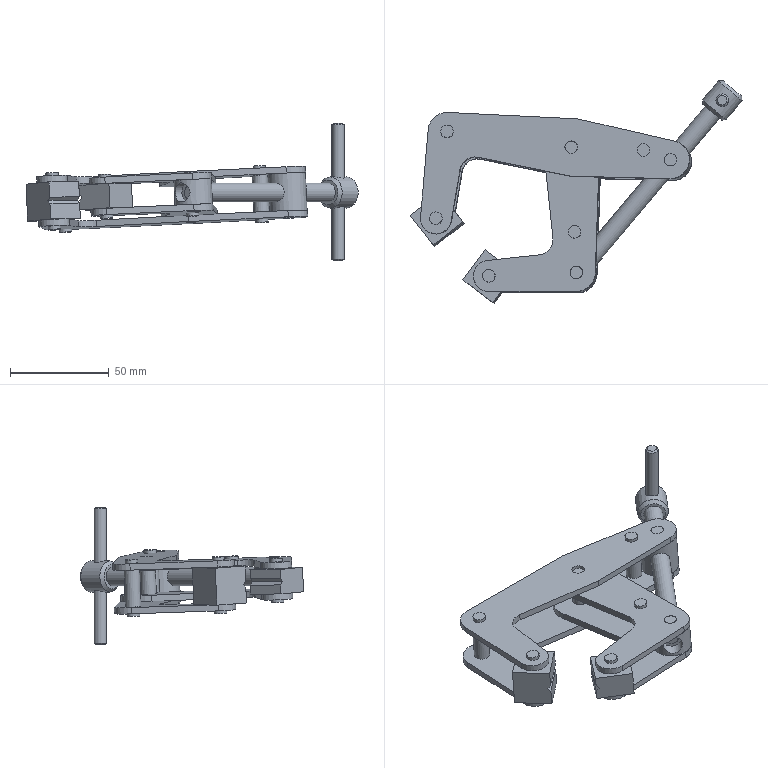Assembly | NX | mm | 16 component files | 16 solids | 158 faces | box 168.42 x 113.11 x 69.85 mm | volume 74950 mm3 | plane 86 | cylinder 68 | cone 4 | commonest cylinder face diameters 6.35 x36 15.748 x9 7.874 x8 19.304 x6 9.525 x2 28.448 x2 7.925 x2 19.05 x2
Bill of materials:
unnamed part 1 | 3 |  | Stepped cylindrical pin: one larger-diameter central body with a smaller coaxial journal at each end.
unnamed part 2 | 1 |  | Roughly cube-shaped rectangular block with a round through hole across one axis and a V-shaped groove running across one side face.
unnamed part 3 | 1 |  | Rectangular block with a round through hole and a single V-shaped notch along one edge face. It looks similar to the other grooved block but with different proportions or groove position.
unnamed part 4 | 2 |  | Flat plate shaped like a dog-leg or L in plan, with rounded ends and five round through holes spread along its arms.
unnamed part 5 | 1 |  | Plain slender solid cylindrical pin or rod with small chamfers at both ends.
unnamed part 6 | 1 |  | Short cylindrical body with one flat cut along its side, a cross hole through it at right angles to the axis, and small coaxial bosses at both ends.
unnamed part 7 | 2 |  | Flat L-shaped plate with rounded ends and corners and four round through holes.
unnamed part 8 | 3 |  | Stepped cylindrical pin with a larger central body and smaller coaxial journals at both ends. It is very similar to the other stepped pin.
unnamed part 9 | 1 |  | Long cylindrical shaft with a larger cylindrical head at one end that has a cross hole through it. The other end steps down to a smaller-diameter tip.
unnamed part 10 | 1 |  | Short cylindrical body with a plain round cross hole through it at right angles to the axis and small coaxial cylindrical bosses at both ends.
Mates:
1. concentric | Riostra_A 2 edge | Riostra_B 2 edge
2. concentric | Pasador_A 3 edge | Riostra_A 2 edge
3. concentric | Pasador_A 2 edge | Riostra_A 2 edge
4. concentric | Articulacion_B 1 edge | Riostra_B 2 edge
5. concentric | Articulacion_A 1 edge | Riostra_A 2 edge
6. concentric | Mordaza_A 1 edge | Riostra_A 2 edge
7. concentric | Riostra_A 2 edge | Pasador_A 1 edge
8. concentric | Mordaza_B 1 edge | Riostra_B 2 edge
9. concentric | Pasador_B 3 edge | Riostra_B 2 edge
10. concentric | Eje 1 edge | Articulacion_B 1 edge
11. touch align | Eje 1 face | Articulacion_A 1 face
12. parallel | Eje 1 face | Articulacion_A 1 face
13. bond | Manivela 1 component | Eje 1 component
14. concentric | Pasador_B 2 edge | Riostra_B 1 edge
15. concentric | Pasador_B 2 edge | Riostra_B 2 edge
16. concentric | Riostra_B 1 edge | Articulacion_B 1 edge
17. concentric | Pasador_B 1 edge | Riostra_B 1 edge
18. concentric | Pasador_B 1 edge | Riostra_B 2 edge
19. concentric | Riostra_A 1 edge | Articulacion_A 1 edge
20. concentric | Riostra_A 1 edge | Pasador_A 3 edge
21. concentric | Riostra_A 1 edge | Riostra_B 1 edge
22. concentric | Riostra_A 1 edge | Pasador_A 2 edge
23. concentric | Pasador_A 1 edge | Riostra_A 1 edge
24. fix | Articulacion_A 1 component